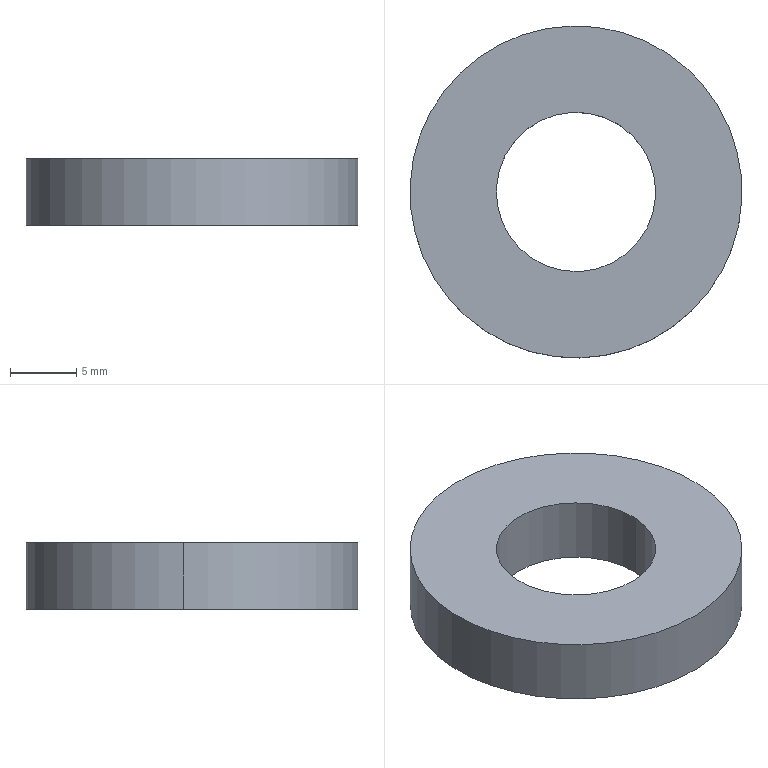Component | SolidWorks | 58-2 | 1 solid | 6 faces | box 25 x 25 x 5 mm | volume 1889 mm3 | cylinder 4 | plane 2 | commonest cylinder face diameters 25 x2 12 x2
build123d program:
from build123d import *

# Parameters (mm, degrees)
SKETCH1_W = 6.5
SKETCH1_H = 5


with BuildPart() as part:
    # Sketch1 → Revolve1 (revolve)
    with BuildSketch(Plane.XY, mode=Mode.PRIVATE) as revolve1_sk:
        with Locations((9.25, 2.5)):
            Rectangle(SKETCH1_W, SKETCH1_H)
    revolve(revolve1_sk.sketch.rotate(Axis((0, 0, 0), (0, 1, 0)), 90), axis=Axis((0, 0, 0), (0, 1, 0)))


solid = part.part

# Placed as in the assembly
solid = solid.moved(Location((0, -38, 356.398), (90, 0, 0)))
STEP:
#1=COLOUR_RGB('',0.7922,0.8196,0.9333);
#2=FILL_AREA_STYLE_COLOUR('',#1);
#3=FILL_AREA_STYLE('',(#2));
#4=SURFACE_STYLE_FILL_AREA(#3);
#5=SURFACE_SIDE_STYLE('',(#4));
#6=SURFACE_STYLE_USAGE(.BOTH.,#5);
#7=PRESENTATION_STYLE_ASSIGNMENT((#6));
#8=CARTESIAN_POINT('',(-0.4915,-1.471,14.228));
#9=VERTEX_POINT('',#8);
#10=CARTESIAN_POINT('',(0.4915,-1.521,14.228));
#11=VERTEX_POINT('',#10);
#12=CARTESIAN_POINT('',(-0.,-1.496,14.228));
#13=DIRECTION('',(-0.,-0.,-1.));
#14=DIRECTION('',(-0.9987,0.05098,0.));
#15=AXIS2_PLACEMENT_3D('',#12,#13,#14);
#16=CIRCLE('',#15,0.4921);
#17=EDGE_CURVE('',#9,#11,#16,.T.);
#18=ORIENTED_EDGE('',*,*,#17,.T.);
#19=CARTESIAN_POINT('',(0.4915,-1.521,14.031));
#20=VERTEX_POINT('',#19);
#21=CARTESIAN_POINT('',(0.4915,-1.521,14.031));
#22=DIRECTION('',(-0.,-0.,-1.));
#23=VECTOR('',#22,39.37);
#24=LINE('',#21,#23);
#25=EDGE_CURVE('',#11,#20,#24,.T.);
#26=ORIENTED_EDGE('',*,*,#25,.T.);
#27=CARTESIAN_POINT('',(-0.4915,-1.471,14.031));
#28=VERTEX_POINT('',#27);
#29=CARTESIAN_POINT('',(-0.,-1.496,14.031));
#30=DIRECTION('',(-0.,-0.,-1.));
#31=DIRECTION('',(-0.9987,0.05098,0.));
#32=AXIS2_PLACEMENT_3D('',#29,#30,#31);
#33=CIRCLE('',#32,0.4921);
#34=EDGE_CURVE('',#28,#20,#33,.T.);
#35=ORIENTED_EDGE('',*,*,#34,.F.);
#36=CARTESIAN_POINT('',(-0.4915,-1.471,14.031));
#37=DIRECTION('',(-0.,-0.,-1.));
#38=VECTOR('',#37,39.37);
#39=LINE('',#36,#38);
#40=EDGE_CURVE('',#9,#28,#39,.T.);
#41=ORIENTED_EDGE('',*,*,#40,.F.);
#42=EDGE_LOOP('',(#18,#26,#35,#41));
#43=FACE_OUTER_BOUND('',#42,.T.);
#44=CARTESIAN_POINT('',(-0.,-1.496,14.031));
#45=DIRECTION('',(-0.,-0.,-1.));
#46=DIRECTION('',(-0.9987,0.05098,0.));
#47=AXIS2_PLACEMENT_3D('',#44,#45,#46);
#48=CYLINDRICAL_SURFACE('',#47,0.4921);
#49=ADVANCED_FACE('',(#43),#48,.T.);
#50=CARTESIAN_POINT('',(0.2359,-1.508,14.228));
#51=VERTEX_POINT('',#50);
#52=CARTESIAN_POINT('',(-0.2359,-1.484,14.228));
#53=VERTEX_POINT('',#52);
#54=CARTESIAN_POINT('',(-0.,-1.496,14.228));
#55=DIRECTION('',(-0.,-0.,-1.));
#56=DIRECTION('',(-0.9987,0.05098,0.));
#57=AXIS2_PLACEMENT_3D('',#54,#55,#56);
#58=CIRCLE('',#57,0.2362);
#59=EDGE_CURVE('',#51,#53,#58,.T.);
#60=ORIENTED_EDGE('',*,*,#59,.F.);
#61=CARTESIAN_POINT('',(0.2359,-1.508,14.031));
#62=VERTEX_POINT('',#61);
#63=CARTESIAN_POINT('',(0.2359,-1.508,14.031));
#64=DIRECTION('',(-0.,-0.,-1.));
#65=VECTOR('',#64,39.37);
#66=LINE('',#63,#65);
#67=EDGE_CURVE('',#51,#62,#66,.T.);
#68=ORIENTED_EDGE('',*,*,#67,.T.);
#69=CARTESIAN_POINT('',(-0.2359,-1.484,14.031));
#70=VERTEX_POINT('',#69);
#71=CARTESIAN_POINT('',(-0.,-1.496,14.031));
#72=DIRECTION('',(-0.,-0.,-1.));
#73=DIRECTION('',(-0.9987,0.05098,0.));
#74=AXIS2_PLACEMENT_3D('',#71,#72,#73);
#75=CIRCLE('',#74,0.2362);
#76=EDGE_CURVE('',#62,#70,#75,.T.);
#77=ORIENTED_EDGE('',*,*,#76,.T.);
#78=CARTESIAN_POINT('',(-0.2359,-1.484,14.031));
#79=DIRECTION('',(-0.,-0.,-1.));
#80=VECTOR('',#79,39.37);
#81=LINE('',#78,#80);
#82=EDGE_CURVE('',#53,#70,#81,.T.);
#83=ORIENTED_EDGE('',*,*,#82,.F.);
#84=EDGE_LOOP('',(#60,#68,#77,#83));
#85=FACE_OUTER_BOUND('',#84,.T.);
#86=CARTESIAN_POINT('',(-0.,-1.496,14.031));
#87=DIRECTION('',(-0.,-0.,-1.));
#88=DIRECTION('',(-0.9987,0.05098,0.));
#89=AXIS2_PLACEMENT_3D('',#86,#87,#88);
#90=CYLINDRICAL_SURFACE('',#89,0.2362);
#91=ADVANCED_FACE('',(#85),#90,.F.);
#92=ORIENTED_EDGE('',*,*,#67,.F.);
#93=CARTESIAN_POINT('',(-0.,-1.496,14.228));
#94=DIRECTION('',(-0.,-0.,-1.));
#95=DIRECTION('',(-0.9987,0.05098,0.));
#96=AXIS2_PLACEMENT_3D('',#93,#94,#95);
#97=CIRCLE('',#96,0.2362);
#98=EDGE_CURVE('',#53,#51,#97,.T.);
#99=ORIENTED_EDGE('',*,*,#98,.F.);
#100=ORIENTED_EDGE('',*,*,#82,.T.);
#101=CARTESIAN_POINT('',(-0.,-1.496,14.031));
#102=DIRECTION('',(-0.,-0.,-1.));
#103=DIRECTION('',(-0.9987,0.05098,0.));
#104=AXIS2_PLACEMENT_3D('',#101,#102,#103);
#105=CIRCLE('',#104,0.2362);
#106=EDGE_CURVE('',#70,#62,#105,.T.);
#107=ORIENTED_EDGE('',*,*,#106,.T.);
#108=EDGE_LOOP('',(#92,#99,#100,#107));
#109=FACE_OUTER_BOUND('',#108,.T.);
#110=CARTESIAN_POINT('',(-0.,-1.496,14.031));
#111=DIRECTION('',(-0.,-0.,-1.));
#112=DIRECTION('',(-0.9987,0.05098,0.));
#113=AXIS2_PLACEMENT_3D('',#110,#111,#112);
#114=CYLINDRICAL_SURFACE('',#113,0.2362);
#115=ADVANCED_FACE('',(#109),#114,.F.);
#116=ORIENTED_EDGE('',*,*,#34,.T.);
#117=CARTESIAN_POINT('',(-0.,-1.496,14.031));
#118=DIRECTION('',(-0.,-0.,-1.));
#119=DIRECTION('',(-0.9987,0.05098,0.));
#120=AXIS2_PLACEMENT_3D('',#117,#118,#119);
#121=CIRCLE('',#120,0.4921);
#122=EDGE_CURVE('',#20,#28,#121,.T.);
#123=ORIENTED_EDGE('',*,*,#122,.T.);
#124=EDGE_LOOP('',(#116,#123));
#125=FACE_OUTER_BOUND('',#124,.T.);
#126=ORIENTED_EDGE('',*,*,#106,.F.);
#127=ORIENTED_EDGE('',*,*,#76,.F.);
#128=EDGE_LOOP('',(#126,#127));
#129=FACE_BOUND('',#128,.T.);
#130=CARTESIAN_POINT('',(0.01204,-1.26,14.031));
#131=DIRECTION('',(-0.,-0.,-1.));
#132=DIRECTION('',(-0.9987,0.05098,-0.));
#133=AXIS2_PLACEMENT_3D('',#130,#131,#132);
#134=PLANE('',#133);
#135=ADVANCED_FACE('',(#125,#129),#134,.T.);
#136=ORIENTED_EDGE('',*,*,#25,.F.);
#137=CARTESIAN_POINT('',(-0.,-1.496,14.228));
#138=DIRECTION('',(-0.,-0.,-1.));
#139=DIRECTION('',(-0.9987,0.05098,0.));
#140=AXIS2_PLACEMENT_3D('',#137,#138,#139);
#141=CIRCLE('',#140,0.4921);
#142=EDGE_CURVE('',#11,#9,#141,.T.);
#143=ORIENTED_EDGE('',*,*,#142,.T.);
#144=ORIENTED_EDGE('',*,*,#40,.T.);
#145=ORIENTED_EDGE('',*,*,#122,.F.);
#146=EDGE_LOOP('',(#136,#143,#144,#145));
#147=FACE_OUTER_BOUND('',#146,.T.);
#148=CARTESIAN_POINT('',(-0.,-1.496,14.031));
#149=DIRECTION('',(-0.,-0.,-1.));
#150=DIRECTION('',(-0.9987,0.05098,0.));
#151=AXIS2_PLACEMENT_3D('',#148,#149,#150);
#152=CYLINDRICAL_SURFACE('',#151,0.4921);
#153=ADVANCED_FACE('',(#147),#152,.T.);
#154=ORIENTED_EDGE('',*,*,#98,.T.);
#155=ORIENTED_EDGE('',*,*,#59,.T.);
#156=EDGE_LOOP('',(#154,#155));
#157=FACE_BOUND('',#156,.T.);
#158=ORIENTED_EDGE('',*,*,#17,.F.);
#159=ORIENTED_EDGE('',*,*,#142,.F.);
#160=EDGE_LOOP('',(#158,#159));
#161=FACE_OUTER_BOUND('',#160,.T.);
#162=CARTESIAN_POINT('',(0.01204,-1.26,14.228));
#163=DIRECTION('',(0.,0.,1.));
#164=DIRECTION('',(0.9987,-0.05098,0.));
#165=AXIS2_PLACEMENT_3D('',#162,#163,#164);
#166=PLANE('',#165);
#167=ADVANCED_FACE('',(#157,#161),#166,.T.);
#168=CLOSED_SHELL('',(#49,#91,#115,#135,#153,#167));
#169=MANIFOLD_SOLID_BREP('',#168);
#170=STYLED_ITEM('',(#7),#169);
#171=PRESENTATION_LAYER_ASSIGNMENT('','',(#170));
#172=(LENGTH_UNIT()NAMED_UNIT(*)SI_UNIT($,.METRE.));
#173=LENGTH_MEASURE_WITH_UNIT(LENGTH_MEASURE(0.0254),#172);
#174=DIMENSIONAL_EXPONENTS(1.,0.,0.,0.,0.,0.,0.);
#175=(CONVERSION_BASED_UNIT('',#173)LENGTH_UNIT()NAMED_UNIT(#174));
#176=UNCERTAINTY_MEASURE_WITH_UNIT(LENGTH_MEASURE(0.00001),#175,'','');
#177=(NAMED_UNIT(*)PLANE_ANGLE_UNIT()SI_UNIT($,.RADIAN.));
#178=(NAMED_UNIT(*)SI_UNIT($,.STERADIAN.)SOLID_ANGLE_UNIT());
#179=(GEOMETRIC_REPRESENTATION_CONTEXT(3)GLOBAL_UNCERTAINTY_ASSIGNED_CONTEXT((#176))GLOBAL_UNIT_ASSIGNED_CONTEXT((#175,#177,#178))REPRESENTATION_CONTEXT('',''));
#180=MECHANICAL_DESIGN_GEOMETRIC_PRESENTATION_REPRESENTATION('',(#170),#179);
#181=CARTESIAN_POINT('',(0.,0.,0.));
#182=DIRECTION('',(0.,0.,1.));
#183=DIRECTION('',(1.,0.,0.));
#184=AXIS2_PLACEMENT_3D('',#181,#182,#183);
#185=(LENGTH_UNIT()NAMED_UNIT(*)SI_UNIT($,.METRE.));
#186=LENGTH_MEASURE_WITH_UNIT(LENGTH_MEASURE(0.0254),#185);
#187=DIMENSIONAL_EXPONENTS(1.,0.,0.,0.,0.,0.,0.);
#188=(CONVERSION_BASED_UNIT('',#186)LENGTH_UNIT()NAMED_UNIT(#187));
#189=UNCERTAINTY_MEASURE_WITH_UNIT(LENGTH_MEASURE(0.00001),#188,'','');
#190=(NAMED_UNIT(*)PLANE_ANGLE_UNIT()SI_UNIT($,.RADIAN.));
#191=(NAMED_UNIT(*)SI_UNIT($,.STERADIAN.)SOLID_ANGLE_UNIT());
#192=(GEOMETRIC_REPRESENTATION_CONTEXT(3)GLOBAL_UNCERTAINTY_ASSIGNED_CONTEXT((#189))GLOBAL_UNIT_ASSIGNED_CONTEXT((#188,#190,#191))REPRESENTATION_CONTEXT('',''));
#193=ADVANCED_BREP_SHAPE_REPRESENTATION('',(#169,#184),#192);